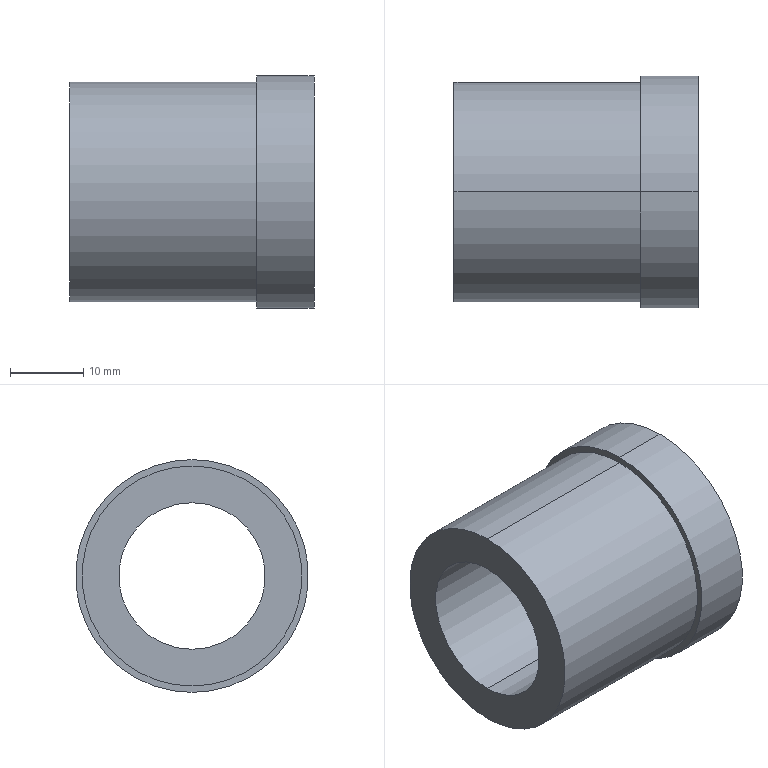Component | SolidWorks | GuideBushingLCHZ20-30-2 | 1 solid | 9 faces | box 33.3 x 31.75 x 31.75 mm | volume 13739 mm3 | cylinder 6 | plane 3 | commonest cylinder face diameters 30 x2 20 x2 31.75 x2
build123d program:
from build123d import *

# Parameters (mm, degrees)
SKETCH1_R           = 15.875
SKETCH1_R_2         = 10
BOSS_EXTRUDE1_DEPTH = 16.65
SKETCH2_OUTSIDE_W   = 44.93
SKETCH2_OUTSIDE_H   = 44.93
SKETCH2_OUTSIDE_R   = 15
CUT_EXTRUDE1_DEPTH  = 25.5


with BuildPart() as part:
    # Sketch1 → Boss-Extrude1 (new, symmetric)
    with BuildSketch(Plane(origin=(0, 0, 0), x_dir=(1, 0, 0), z_dir=(0, 1, 0))):
        with Locations(Location((0, 0, 0), (0, 0, 270))):
            Circle(SKETCH1_R)
        with Locations(Location((0, 0, 0), (0, 0, 270))):
            Circle(SKETCH1_R_2, mode=Mode.SUBTRACT)
    extrude(amount=BOSS_EXTRUDE1_DEPTH, both=True)

    # Sketch2 outside → Cut-Extrude1 (cut)
    with BuildSketch(Plane(origin=(0, 16.65, 0), x_dir=(1, 0, 0), z_dir=(0, 1, 0))):
        Rectangle(SKETCH2_OUTSIDE_W, SKETCH2_OUTSIDE_H)
        with Locations(Location((0, 0, 0), (0, 0, 270))):
            Circle(SKETCH2_OUTSIDE_R, mode=Mode.SUBTRACT)
    extrude(amount=-CUT_EXTRUDE1_DEPTH, mode=Mode.SUBTRACT)


solid = part.part

# Placed as in the assembly
solid = solid.moved(Location((394.542, 317.499, 103), (0, 0, 90)))
STEP:
#1=COLOUR_RGB('',0.7922,0.8196,0.9333);
#2=FILL_AREA_STYLE_COLOUR('',#1);
#3=FILL_AREA_STYLE('',(#2));
#4=SURFACE_STYLE_FILL_AREA(#3);
#5=SURFACE_SIDE_STYLE('',(#4));
#6=SURFACE_STYLE_USAGE(.BOTH.,#5);
#7=PRESENTATION_STYLE_ASSIGNMENT((#6));
#8=CARTESIAN_POINT('',(15.882,12.5,4.646));
#9=VERTEX_POINT('',#8);
#10=CARTESIAN_POINT('',(15.882,12.5,3.465));
#11=VERTEX_POINT('',#10);
#12=CARTESIAN_POINT('',(15.882,12.5,4.055));
#13=DIRECTION('',(-1.,0.,-0.));
#14=DIRECTION('',(0.,0.,1.));
#15=AXIS2_PLACEMENT_3D('',#12,#13,#14);
#16=CIRCLE('',#15,0.5906);
#17=EDGE_CURVE('',#9,#11,#16,.T.);
#18=ORIENTED_EDGE('',*,*,#17,.T.);
#19=CARTESIAN_POINT('',(14.878,12.5,3.465));
#20=VERTEX_POINT('',#19);
#21=CARTESIAN_POINT('',(15.882,12.5,3.465));
#22=DIRECTION('',(-1.,0.,-0.));
#23=VECTOR('',#22,39.37);
#24=LINE('',#21,#23);
#25=EDGE_CURVE('',#11,#20,#24,.T.);
#26=ORIENTED_EDGE('',*,*,#25,.T.);
#27=CARTESIAN_POINT('',(14.878,12.5,4.646));
#28=VERTEX_POINT('',#27);
#29=CARTESIAN_POINT('',(14.878,12.5,4.055));
#30=DIRECTION('',(-1.,0.,-0.));
#31=DIRECTION('',(0.,0.,1.));
#32=AXIS2_PLACEMENT_3D('',#29,#30,#31);
#33=CIRCLE('',#32,0.5906);
#34=EDGE_CURVE('',#28,#20,#33,.T.);
#35=ORIENTED_EDGE('',*,*,#34,.F.);
#36=CARTESIAN_POINT('',(15.882,12.5,4.646));
#37=DIRECTION('',(-1.,0.,-0.));
#38=VECTOR('',#37,39.37);
#39=LINE('',#36,#38);
#40=EDGE_CURVE('',#9,#28,#39,.T.);
#41=ORIENTED_EDGE('',*,*,#40,.F.);
#42=EDGE_LOOP('',(#18,#26,#35,#41));
#43=FACE_OUTER_BOUND('',#42,.T.);
#44=CARTESIAN_POINT('',(15.882,12.5,4.055));
#45=DIRECTION('',(-1.,0.,-0.));
#46=DIRECTION('',(0.,0.,1.));
#47=AXIS2_PLACEMENT_3D('',#44,#45,#46);
#48=CYLINDRICAL_SURFACE('',#47,0.5906);
#49=ADVANCED_FACE('',(#43),#48,.T.);
#50=CARTESIAN_POINT('',(14.878,12.5,3.661));
#51=VERTEX_POINT('',#50);
#52=CARTESIAN_POINT('',(14.878,12.5,4.449));
#53=VERTEX_POINT('',#52);
#54=CARTESIAN_POINT('',(14.878,12.5,4.055));
#55=DIRECTION('',(-1.,0.,-0.));
#56=DIRECTION('',(0.,0.,1.));
#57=AXIS2_PLACEMENT_3D('',#54,#55,#56);
#58=CIRCLE('',#57,0.3937);
#59=EDGE_CURVE('',#51,#53,#58,.T.);
#60=ORIENTED_EDGE('',*,*,#59,.T.);
#61=CARTESIAN_POINT('',(16.189,12.5,4.449));
#62=VERTEX_POINT('',#61);
#63=CARTESIAN_POINT('',(14.878,12.5,4.449));
#64=DIRECTION('',(1.,-0.,0.));
#65=VECTOR('',#64,39.37);
#66=LINE('',#63,#65);
#67=EDGE_CURVE('',#53,#62,#66,.T.);
#68=ORIENTED_EDGE('',*,*,#67,.T.);
#69=CARTESIAN_POINT('',(16.189,12.5,3.661));
#70=VERTEX_POINT('',#69);
#71=CARTESIAN_POINT('',(16.189,12.5,4.055));
#72=DIRECTION('',(-1.,0.,-0.));
#73=DIRECTION('',(0.,0.,1.));
#74=AXIS2_PLACEMENT_3D('',#71,#72,#73);
#75=CIRCLE('',#74,0.3937);
#76=EDGE_CURVE('',#70,#62,#75,.T.);
#77=ORIENTED_EDGE('',*,*,#76,.F.);
#78=CARTESIAN_POINT('',(14.878,12.5,3.661));
#79=DIRECTION('',(1.,-0.,0.));
#80=VECTOR('',#79,39.37);
#81=LINE('',#78,#80);
#82=EDGE_CURVE('',#51,#70,#81,.T.);
#83=ORIENTED_EDGE('',*,*,#82,.F.);
#84=EDGE_LOOP('',(#60,#68,#77,#83));
#85=FACE_OUTER_BOUND('',#84,.T.);
#86=CARTESIAN_POINT('',(14.878,12.5,4.055));
#87=DIRECTION('',(1.,-0.,0.));
#88=DIRECTION('',(0.,0.,-1.));
#89=AXIS2_PLACEMENT_3D('',#86,#87,#88);
#90=CYLINDRICAL_SURFACE('',#89,0.3937);
#91=ADVANCED_FACE('',(#85),#90,.F.);
#92=CARTESIAN_POINT('',(15.882,12.5,4.68));
#93=VERTEX_POINT('',#92);
#94=CARTESIAN_POINT('',(15.882,12.5,3.43));
#95=VERTEX_POINT('',#94);
#96=CARTESIAN_POINT('',(15.882,12.5,4.055));
#97=DIRECTION('',(-1.,0.,-0.));
#98=DIRECTION('',(0.,0.,1.));
#99=AXIS2_PLACEMENT_3D('',#96,#97,#98);
#100=CIRCLE('',#99,0.625);
#101=EDGE_CURVE('',#93,#95,#100,.T.);
#102=ORIENTED_EDGE('',*,*,#101,.F.);
#103=CARTESIAN_POINT('',(16.189,12.5,4.68));
#104=VERTEX_POINT('',#103);
#105=CARTESIAN_POINT('',(14.878,12.5,4.68));
#106=DIRECTION('',(1.,-0.,0.));
#107=VECTOR('',#106,39.37);
#108=LINE('',#105,#107);
#109=EDGE_CURVE('',#93,#104,#108,.T.);
#110=ORIENTED_EDGE('',*,*,#109,.T.);
#111=CARTESIAN_POINT('',(16.189,12.5,3.43));
#112=VERTEX_POINT('',#111);
#113=CARTESIAN_POINT('',(16.189,12.5,4.055));
#114=DIRECTION('',(-1.,0.,-0.));
#115=DIRECTION('',(0.,0.,1.));
#116=AXIS2_PLACEMENT_3D('',#113,#114,#115);
#117=CIRCLE('',#116,0.625);
#118=EDGE_CURVE('',#104,#112,#117,.T.);
#119=ORIENTED_EDGE('',*,*,#118,.T.);
#120=CARTESIAN_POINT('',(14.878,12.5,3.43));
#121=DIRECTION('',(1.,-0.,0.));
#122=VECTOR('',#121,39.37);
#123=LINE('',#120,#122);
#124=EDGE_CURVE('',#95,#112,#123,.T.);
#125=ORIENTED_EDGE('',*,*,#124,.F.);
#126=EDGE_LOOP('',(#102,#110,#119,#125));
#127=FACE_OUTER_BOUND('',#126,.T.);
#128=CARTESIAN_POINT('',(14.878,12.5,4.055));
#129=DIRECTION('',(1.,-0.,0.));
#130=DIRECTION('',(0.,0.,-1.));
#131=AXIS2_PLACEMENT_3D('',#128,#129,#130);
#132=CYLINDRICAL_SURFACE('',#131,0.625);
#133=ADVANCED_FACE('',(#127),#132,.T.);
#134=ORIENTED_EDGE('',*,*,#59,.F.);
#135=CARTESIAN_POINT('',(14.878,12.5,4.055));
#136=DIRECTION('',(-1.,0.,-0.));
#137=DIRECTION('',(0.,0.,1.));
#138=AXIS2_PLACEMENT_3D('',#135,#136,#137);
#139=CIRCLE('',#138,0.3937);
#140=EDGE_CURVE('',#53,#51,#139,.T.);
#141=ORIENTED_EDGE('',*,*,#140,.F.);
#142=EDGE_LOOP('',(#134,#141));
#143=FACE_BOUND('',#142,.T.);
#144=ORIENTED_EDGE('',*,*,#34,.T.);
#145=CARTESIAN_POINT('',(14.878,12.5,4.055));
#146=DIRECTION('',(-1.,0.,-0.));
#147=DIRECTION('',(0.,0.,1.));
#148=AXIS2_PLACEMENT_3D('',#145,#146,#147);
#149=CIRCLE('',#148,0.5906);
#150=EDGE_CURVE('',#20,#28,#149,.T.);
#151=ORIENTED_EDGE('',*,*,#150,.T.);
#152=EDGE_LOOP('',(#144,#151));
#153=FACE_OUTER_BOUND('',#152,.T.);
#154=CARTESIAN_POINT('',(14.878,12.5,4.055));
#155=DIRECTION('',(-1.,0.,0.));
#156=DIRECTION('',(0.,-0.,1.));
#157=AXIS2_PLACEMENT_3D('',#154,#155,#156);
#158=PLANE('',#157);
#159=ADVANCED_FACE('',(#143,#153),#158,.T.);
#160=ORIENTED_EDGE('',*,*,#109,.F.);
#161=CARTESIAN_POINT('',(15.882,12.5,4.055));
#162=DIRECTION('',(-1.,0.,-0.));
#163=DIRECTION('',(0.,0.,1.));
#164=AXIS2_PLACEMENT_3D('',#161,#162,#163);
#165=CIRCLE('',#164,0.625);
#166=EDGE_CURVE('',#95,#93,#165,.T.);
#167=ORIENTED_EDGE('',*,*,#166,.F.);
#168=ORIENTED_EDGE('',*,*,#124,.T.);
#169=CARTESIAN_POINT('',(16.189,12.5,4.055));
#170=DIRECTION('',(-1.,0.,-0.));
#171=DIRECTION('',(0.,0.,1.));
#172=AXIS2_PLACEMENT_3D('',#169,#170,#171);
#173=CIRCLE('',#172,0.625);
#174=EDGE_CURVE('',#112,#104,#173,.T.);
#175=ORIENTED_EDGE('',*,*,#174,.T.);
#176=EDGE_LOOP('',(#160,#167,#168,#175));
#177=FACE_OUTER_BOUND('',#176,.T.);
#178=CARTESIAN_POINT('',(14.878,12.5,4.055));
#179=DIRECTION('',(1.,-0.,0.));
#180=DIRECTION('',(0.,0.,-1.));
#181=AXIS2_PLACEMENT_3D('',#178,#179,#180);
#182=CYLINDRICAL_SURFACE('',#181,0.625);
#183=ADVANCED_FACE('',(#177),#182,.T.);
#184=ORIENTED_EDGE('',*,*,#174,.F.);
#185=ORIENTED_EDGE('',*,*,#118,.F.);
#186=EDGE_LOOP('',(#184,#185));
#187=FACE_OUTER_BOUND('',#186,.T.);
#188=ORIENTED_EDGE('',*,*,#76,.T.);
#189=CARTESIAN_POINT('',(16.189,12.5,4.055));
#190=DIRECTION('',(-1.,0.,-0.));
#191=DIRECTION('',(0.,0.,1.));
#192=AXIS2_PLACEMENT_3D('',#189,#190,#191);
#193=CIRCLE('',#192,0.3937);
#194=EDGE_CURVE('',#62,#70,#193,.T.);
#195=ORIENTED_EDGE('',*,*,#194,.T.);
#196=EDGE_LOOP('',(#188,#195));
#197=FACE_BOUND('',#196,.T.);
#198=CARTESIAN_POINT('',(16.189,12.5,4.055));
#199=DIRECTION('',(-1.,0.,0.));
#200=DIRECTION('',(0.,-0.,1.));
#201=AXIS2_PLACEMENT_3D('',#198,#199,#200);
#202=PLANE('',#201);
#203=ADVANCED_FACE('',(#187,#197),#202,.F.);
#204=ORIENTED_EDGE('',*,*,#67,.F.);
#205=ORIENTED_EDGE('',*,*,#140,.T.);
#206=ORIENTED_EDGE('',*,*,#82,.T.);
#207=ORIENTED_EDGE('',*,*,#194,.F.);
#208=EDGE_LOOP('',(#204,#205,#206,#207));
#209=FACE_OUTER_BOUND('',#208,.T.);
#210=CARTESIAN_POINT('',(14.878,12.5,4.055));
#211=DIRECTION('',(1.,-0.,0.));
#212=DIRECTION('',(0.,0.,-1.));
#213=AXIS2_PLACEMENT_3D('',#210,#211,#212);
#214=CYLINDRICAL_SURFACE('',#213,0.3937);
#215=ADVANCED_FACE('',(#209),#214,.F.);
#216=ORIENTED_EDGE('',*,*,#17,.F.);
#217=CARTESIAN_POINT('',(15.882,12.5,4.055));
#218=DIRECTION('',(-1.,0.,-0.));
#219=DIRECTION('',(0.,0.,1.));
#220=AXIS2_PLACEMENT_3D('',#217,#218,#219);
#221=CIRCLE('',#220,0.5906);
#222=EDGE_CURVE('',#11,#9,#221,.T.);
#223=ORIENTED_EDGE('',*,*,#222,.F.);
#224=EDGE_LOOP('',(#216,#223));
#225=FACE_BOUND('',#224,.T.);
#226=ORIENTED_EDGE('',*,*,#166,.T.);
#227=ORIENTED_EDGE('',*,*,#101,.T.);
#228=EDGE_LOOP('',(#226,#227));
#229=FACE_OUTER_BOUND('',#228,.T.);
#230=CARTESIAN_POINT('',(15.882,12.5,4.055));
#231=DIRECTION('',(-1.,0.,0.));
#232=DIRECTION('',(0.,-0.,1.));
#233=AXIS2_PLACEMENT_3D('',#230,#231,#232);
#234=PLANE('',#233);
#235=ADVANCED_FACE('',(#225,#229),#234,.T.);
#236=ORIENTED_EDGE('',*,*,#25,.F.);
#237=ORIENTED_EDGE('',*,*,#222,.T.);
#238=ORIENTED_EDGE('',*,*,#40,.T.);
#239=ORIENTED_EDGE('',*,*,#150,.F.);
#240=EDGE_LOOP('',(#236,#237,#238,#239));
#241=FACE_OUTER_BOUND('',#240,.T.);
#242=CARTESIAN_POINT('',(15.882,12.5,4.055));
#243=DIRECTION('',(-1.,0.,-0.));
#244=DIRECTION('',(0.,0.,1.));
#245=AXIS2_PLACEMENT_3D('',#242,#243,#244);
#246=CYLINDRICAL_SURFACE('',#245,0.5906);
#247=ADVANCED_FACE('',(#241),#246,.T.);
#248=CLOSED_SHELL('',(#49,#91,#133,#159,#183,#203,#215,#235,#247));
#249=MANIFOLD_SOLID_BREP('',#248);
#250=STYLED_ITEM('',(#7),#249);
#251=(LENGTH_UNIT()NAMED_UNIT(*)SI_UNIT($,.METRE.));
#252=LENGTH_MEASURE_WITH_UNIT(LENGTH_MEASURE(0.0254),#251);
#253=DIMENSIONAL_EXPONENTS(1.,0.,0.,0.,0.,0.,0.);
#254=(CONVERSION_BASED_UNIT('',#252)LENGTH_UNIT()NAMED_UNIT(#253));
#255=UNCERTAINTY_MEASURE_WITH_UNIT(LENGTH_MEASURE(0.00001),#254,'','');
#256=(NAMED_UNIT(*)PLANE_ANGLE_UNIT()SI_UNIT($,.RADIAN.));
#257=(NAMED_UNIT(*)SI_UNIT($,.STERADIAN.)SOLID_ANGLE_UNIT());
#258=(GEOMETRIC_REPRESENTATION_CONTEXT(3)GLOBAL_UNCERTAINTY_ASSIGNED_CONTEXT((#255))GLOBAL_UNIT_ASSIGNED_CONTEXT((#254,#256,#257))REPRESENTATION_CONTEXT('',''));
#259=MECHANICAL_DESIGN_GEOMETRIC_PRESENTATION_REPRESENTATION('',(#250),#258);
#260=CARTESIAN_POINT('',(0.,0.,0.));
#261=DIRECTION('',(0.,0.,1.));
#262=DIRECTION('',(1.,0.,0.));
#263=AXIS2_PLACEMENT_3D('',#260,#261,#262);
#264=(LENGTH_UNIT()NAMED_UNIT(*)SI_UNIT($,.METRE.));
#265=LENGTH_MEASURE_WITH_UNIT(LENGTH_MEASURE(0.0254),#264);
#266=DIMENSIONAL_EXPONENTS(1.,0.,0.,0.,0.,0.,0.);
#267=(CONVERSION_BASED_UNIT('',#265)LENGTH_UNIT()NAMED_UNIT(#266));
#268=UNCERTAINTY_MEASURE_WITH_UNIT(LENGTH_MEASURE(0.00001),#267,'','');
#269=(NAMED_UNIT(*)PLANE_ANGLE_UNIT()SI_UNIT($,.RADIAN.));
#270=(NAMED_UNIT(*)SI_UNIT($,.STERADIAN.)SOLID_ANGLE_UNIT());
#271=(GEOMETRIC_REPRESENTATION_CONTEXT(3)GLOBAL_UNCERTAINTY_ASSIGNED_CONTEXT((#268))GLOBAL_UNIT_ASSIGNED_CONTEXT((#267,#269,#270))REPRESENTATION_CONTEXT('',''));
#272=ADVANCED_BREP_SHAPE_REPRESENTATION('',(#249,#263),#271);
#273=PRESENTATION_LAYER_ASSIGNMENT('','',(#250));